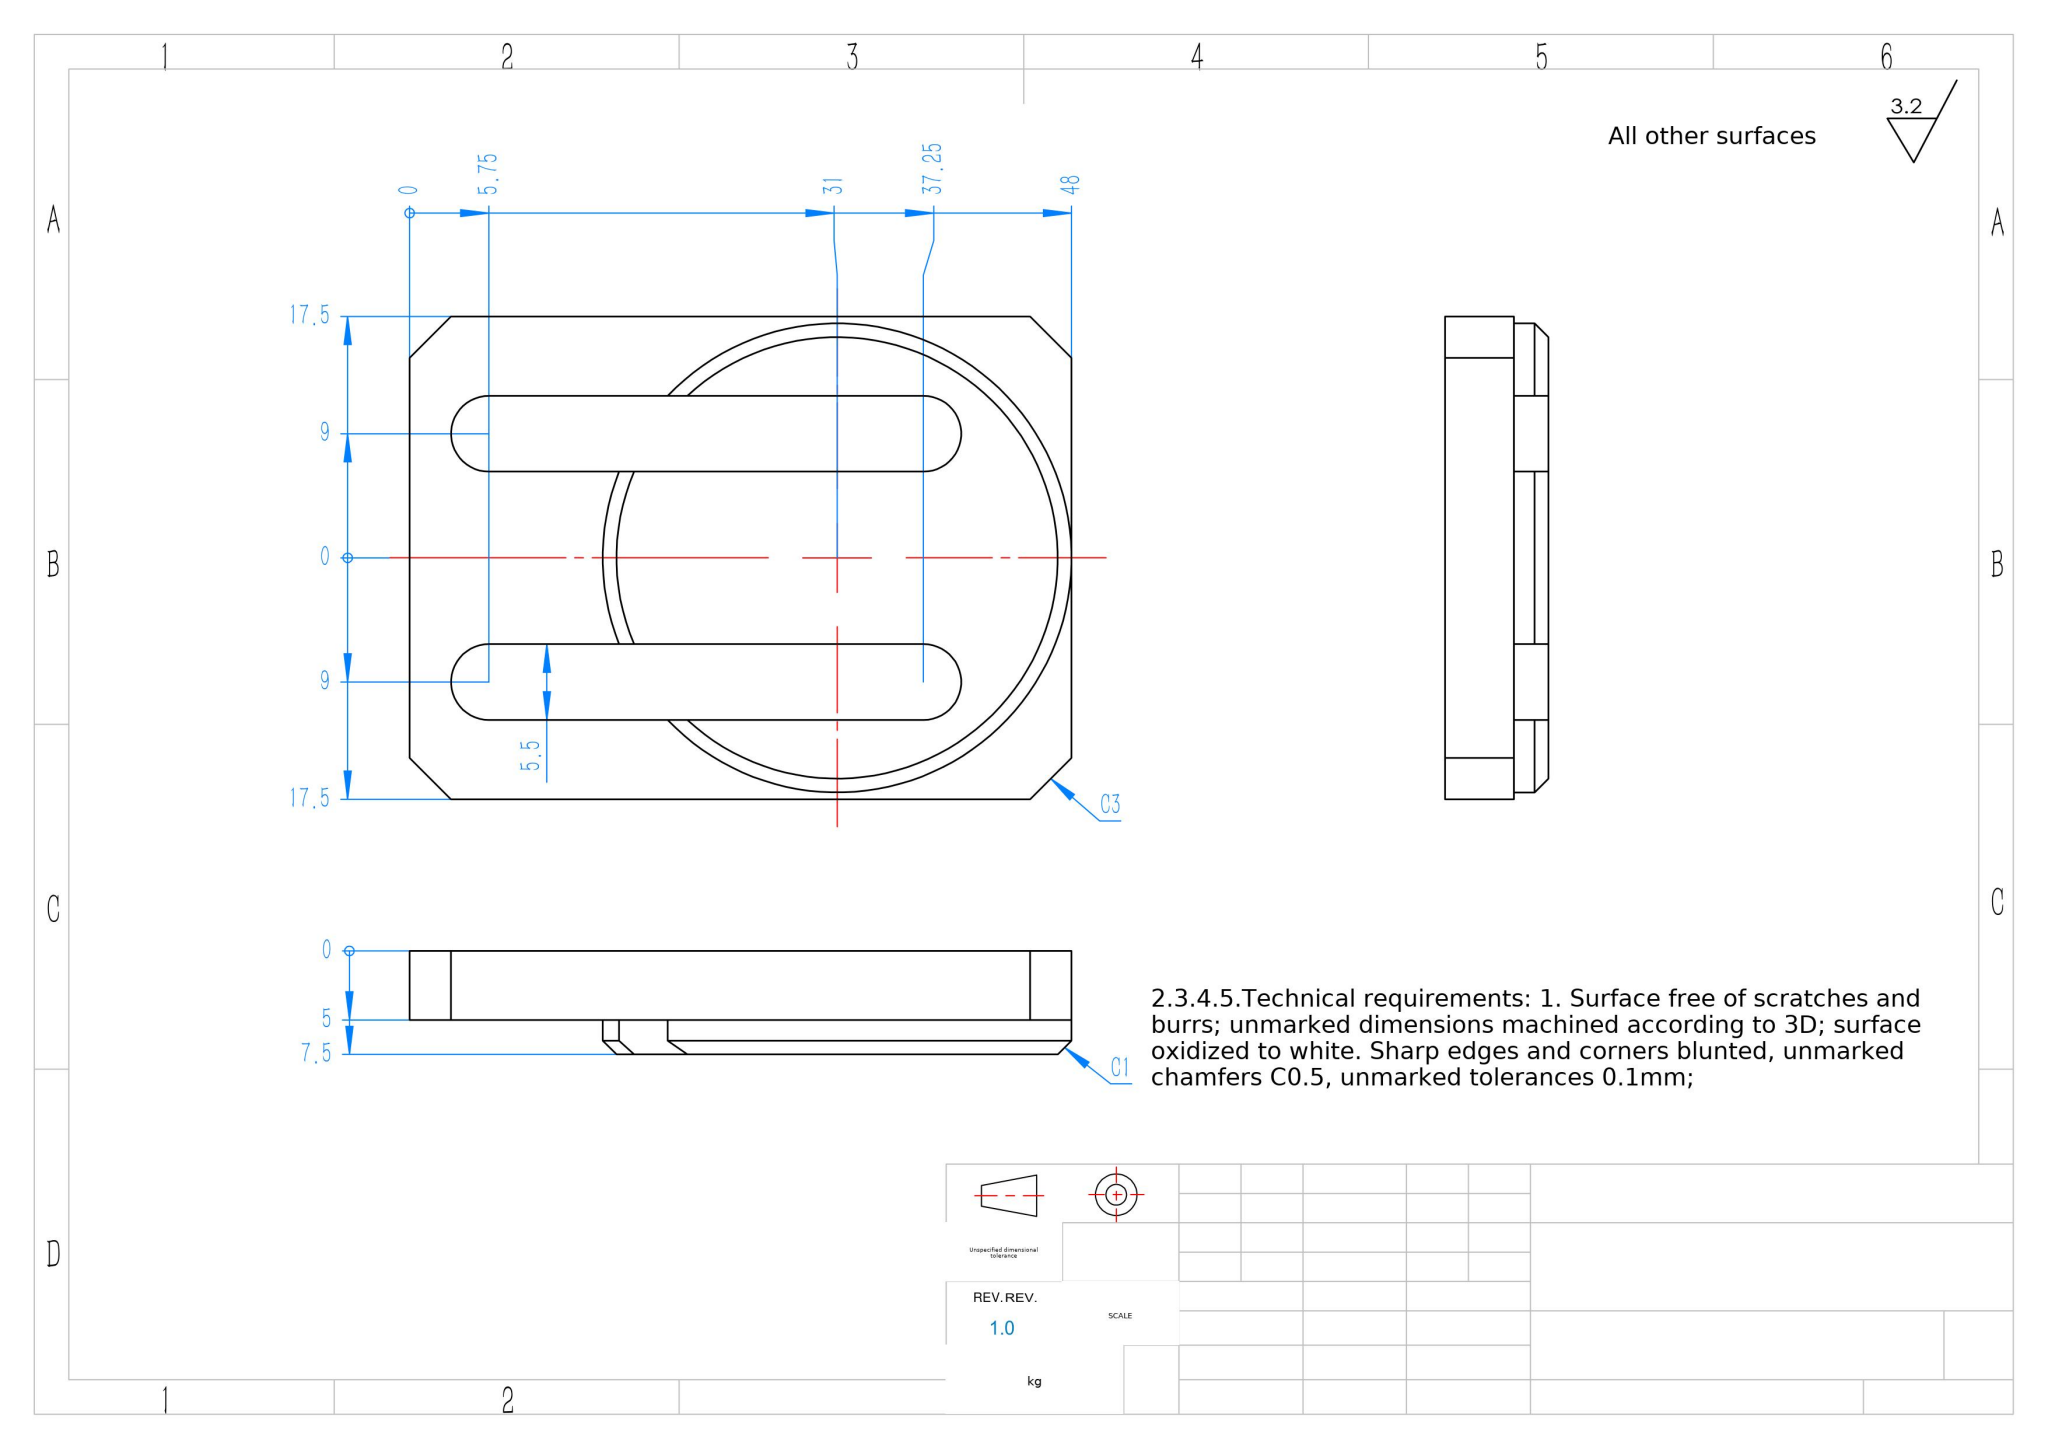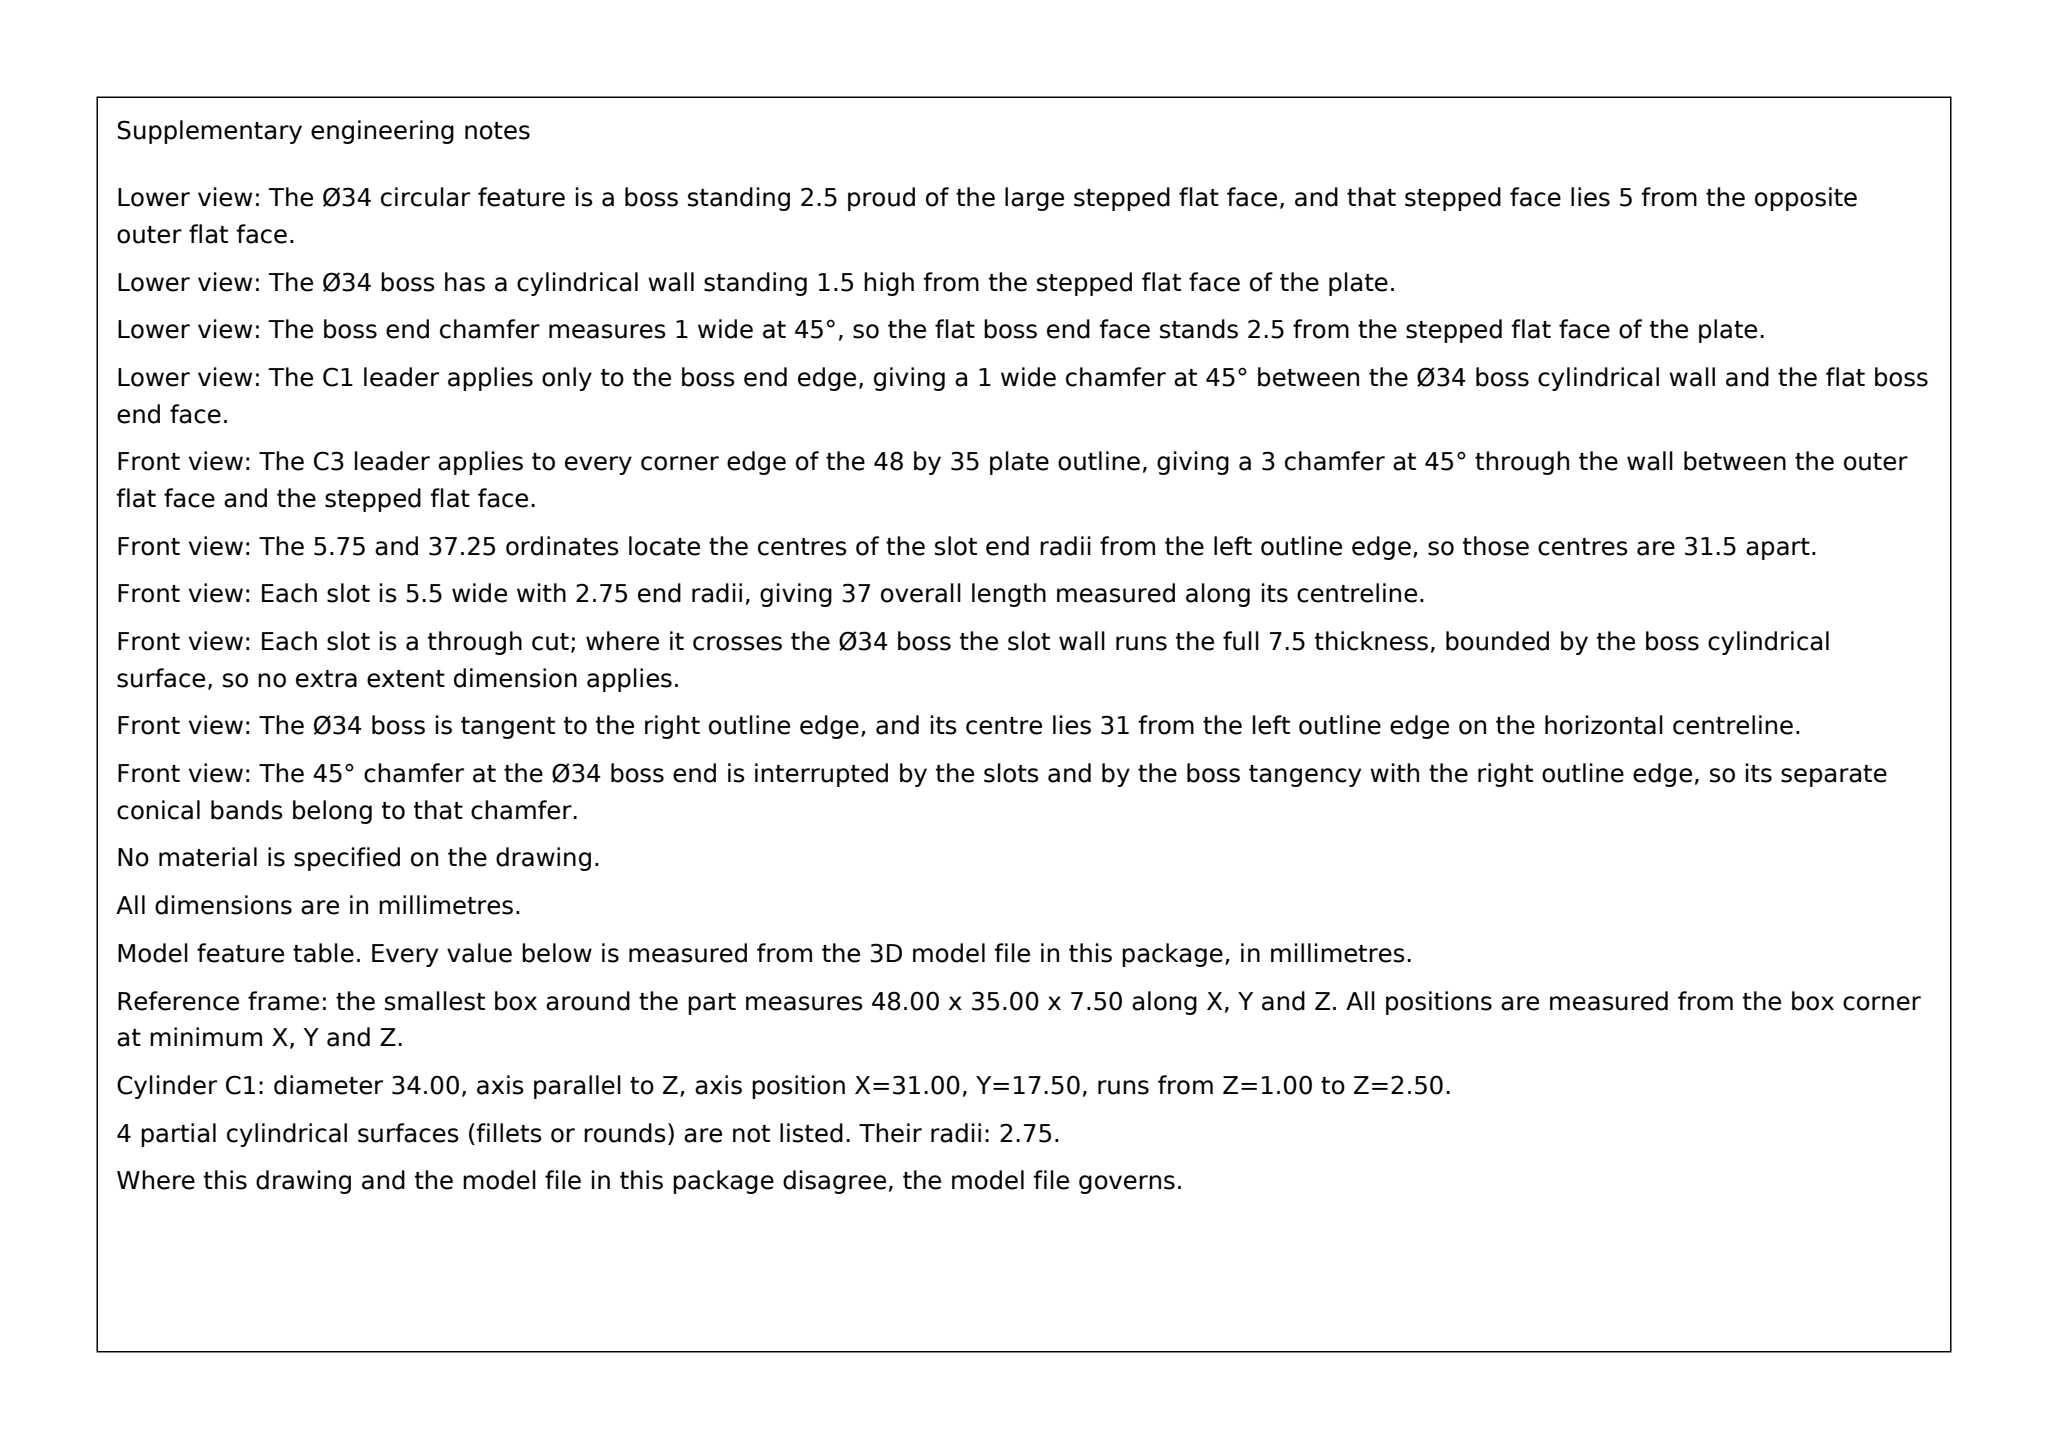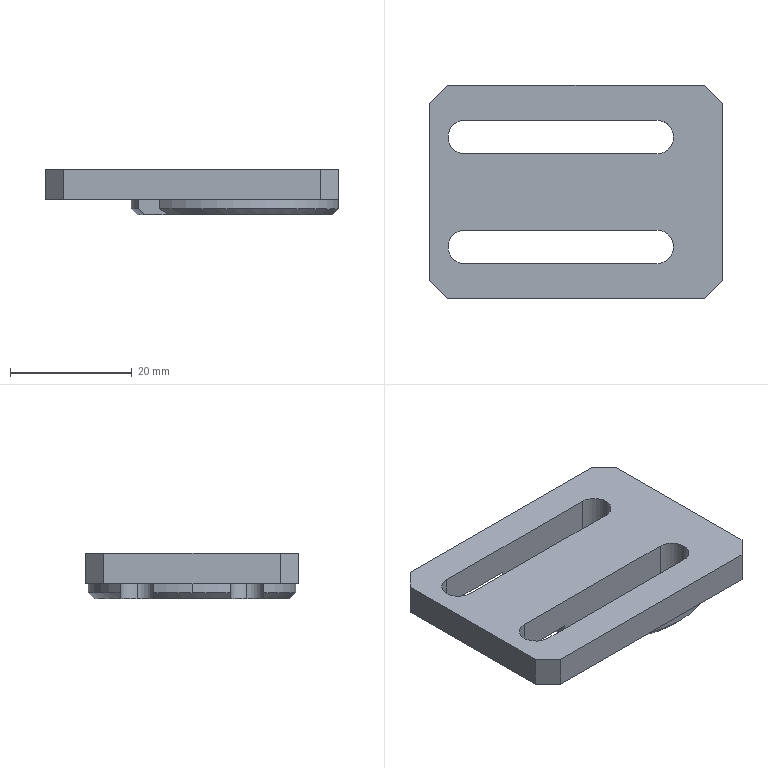Part | SolidWorks | mm | 1 solid | 27 faces | box 48 x 35 x 7.5 mm | volume 7940 mm3 | plane 15 | cylinder 9 | cone 3 | commonest cylinder face diameters 5.5 x6 34 x3
Drawing notes:
Ø34 RECESS DP 1.5 FROM BOTTOM FACE (7.5 SIDE) | from the solid: cyl dia34 axis z at (31,17.5), length 1.5, spans z0-1.5 of 7.5 thk
Ø34 RECESS ENTRY 90° INCL CSK FORM, MACHINED FROM BOTTOM FACE | from the solid: cones[included_angle,ref_dia]=[90.0,34.0]; z=0 face side
SLOTS 5 DP FROM TOP FACE, FLOOR 2.5 ABOVE BTM; THRU AT 37.25 END | from the solid: Ø5.5 cyls len 5.0 at x5.75, len 7.5 at x37.25; z-plane at 2.5
SLOT ENDS R2.75 (1/2 OF 5.5 W), CL AT X=5.75 & X=37.25 | from the solid: Ø5.5 cyls at x5.75/37.25, y8.5 & 26.5; slot width 5.5
Ø34 DP 1.5 W/ 90° CSK TO Ø37 AT BOTTOM FACE | from the solid: cylinder dia 34 z-axis at (31,17.5) len 1.5; cone incl angle 90° ref dia 34 -> 34+2(1.5)=Ø37 at z=7.5 face